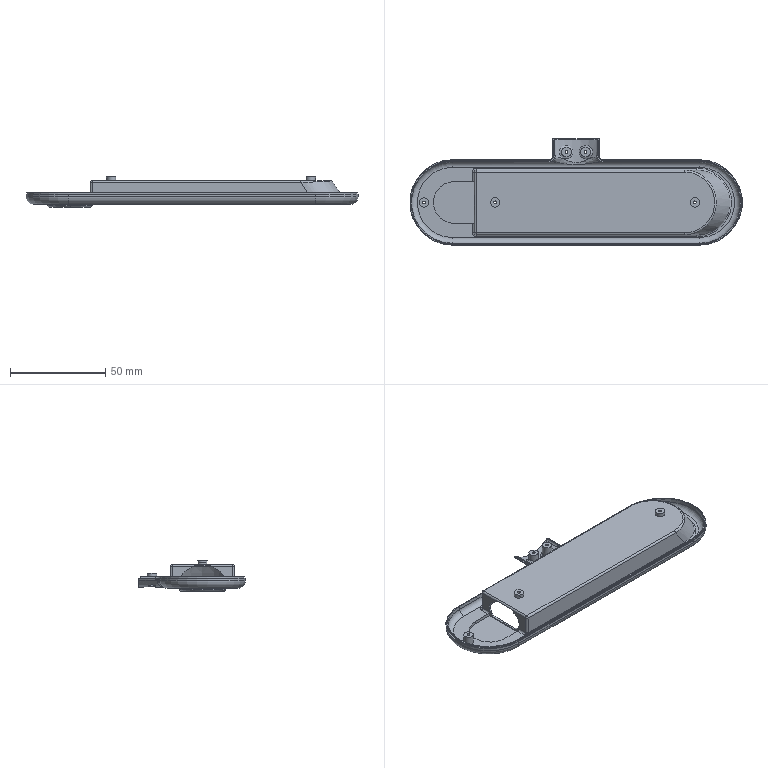Component | NX | XIADENGKE | 1 solid | 134 faces | volume 12182 mm3 | cylinder 55 | plane 44 | spline 17 | torus 13 | cone 3 | sphere 2 | commonest cylinder face diameters 2 x11 4 x9 5 x9 1.5 x5 10 x2 8 x2 6 x2 45 x2